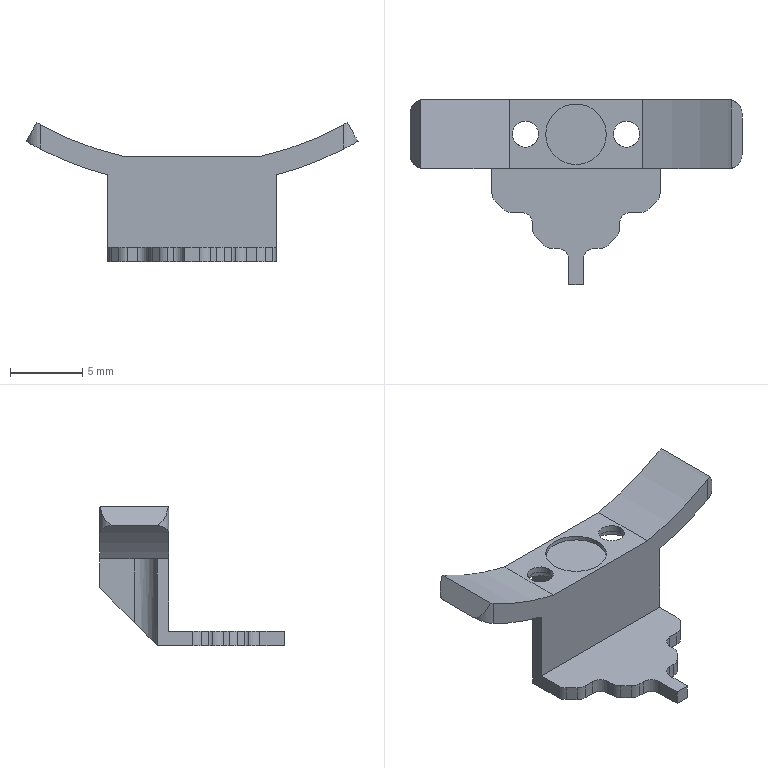CAM job | Mastercam | mm | 23 operations | part box 23 x 12.8 x 9.63
1. 3D High Speed (Dynamic OptiRough) | 2 - 10C
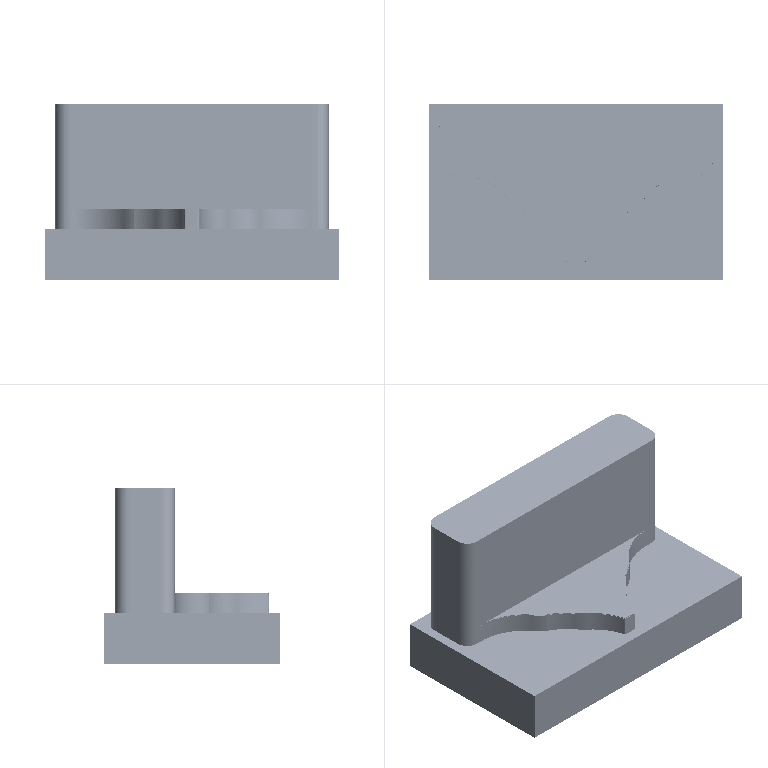2. Contour (2D) | 3 - 10J
3. Contour (2D) | 3 - 10J
4. Contour (2D) | 5 - 4J
5. Contour (Ramp) | 27 - 3 平铣刀
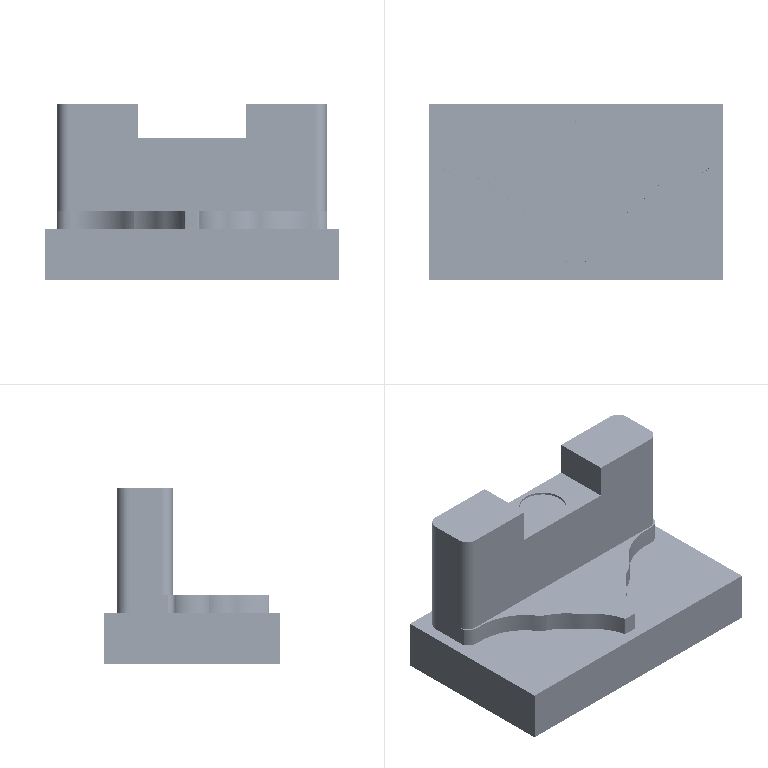6. Contour (2D) | 27 - 3 平铣刀
7. Contour (Ramp) | 16 - 1 平铣刀
8. Contour (2D) | 16 - 1 平铣刀
9. Surface Finish Flowline | 15 - 4 圆鼻铣刀
10. Surface Finish Flowline | 15 - 4 圆鼻铣刀
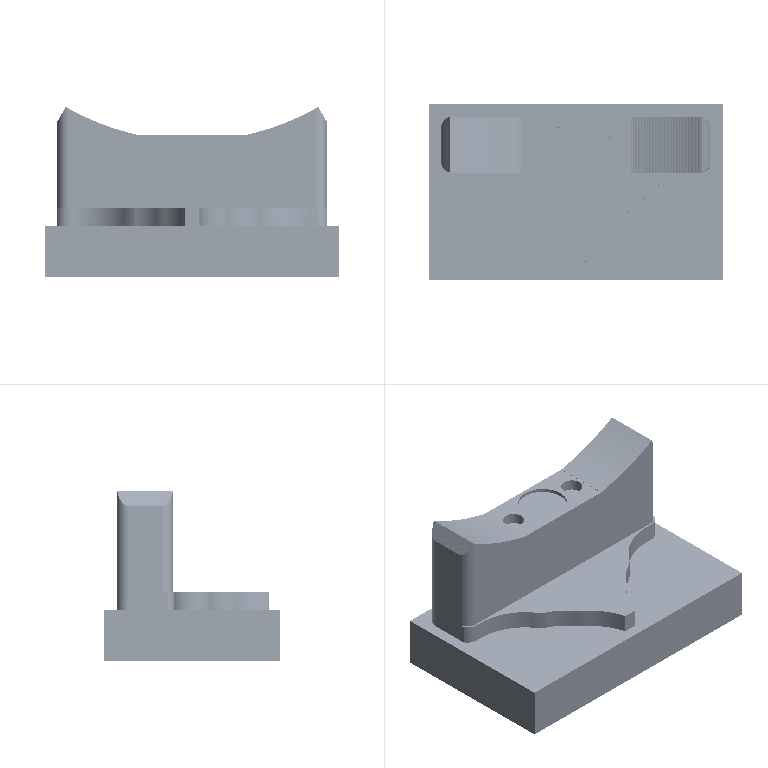11. Facing | 2 - 10C
12. 3D High Speed (Area rest roughing) | 4 - 4C
13. Facing | 5 - 4J
14. Contour (2D) | 5 - 4J
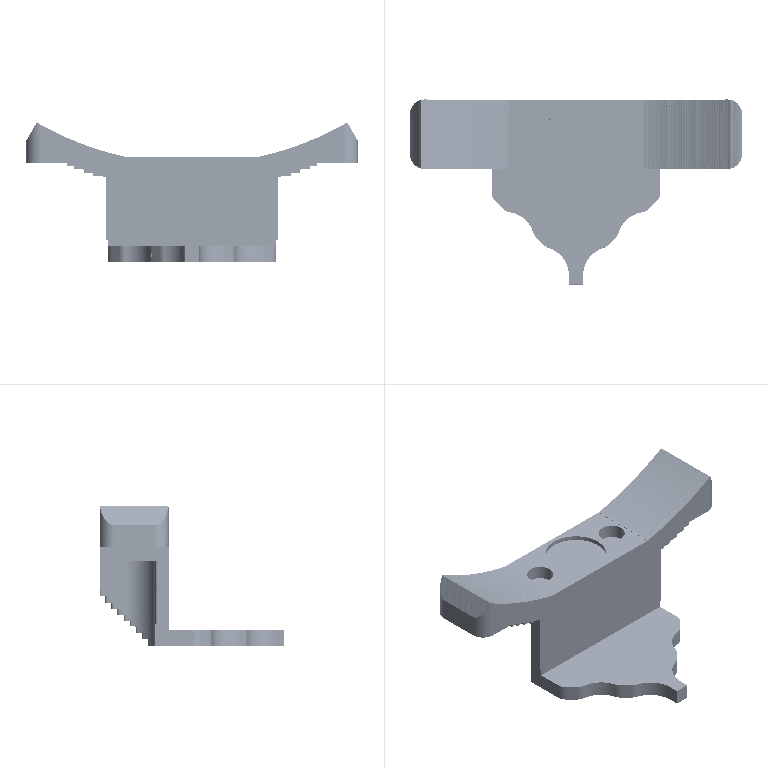15. Contour (2D) | 5 - 4J
16. Contour (2D) | 5 - 4J
17. Contour (Ramp) | 12 - 2C
18. Contour (2D) | 13 - 2J
19. Contour (Remachining) | 16 - 1 平铣刀
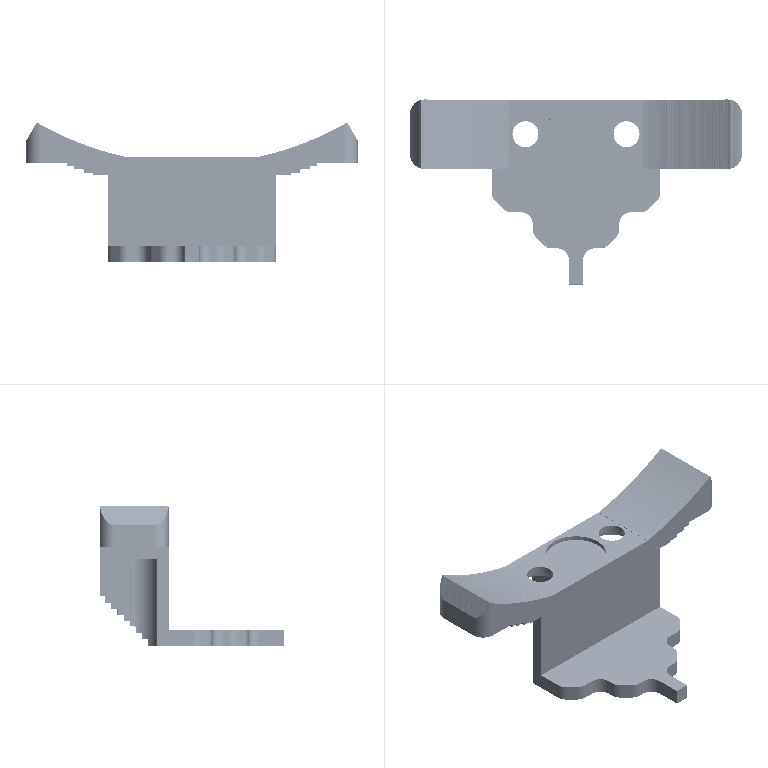20. Surface Finish Flowline | 15 - 4 圆鼻铣刀
21. Surface Finish Flowline | 15 - 4 圆鼻铣刀
22. Surface Finish Flowline | 15 - 4 圆鼻铣刀
23. Model Chamfer | 6 - 6 倒角刀